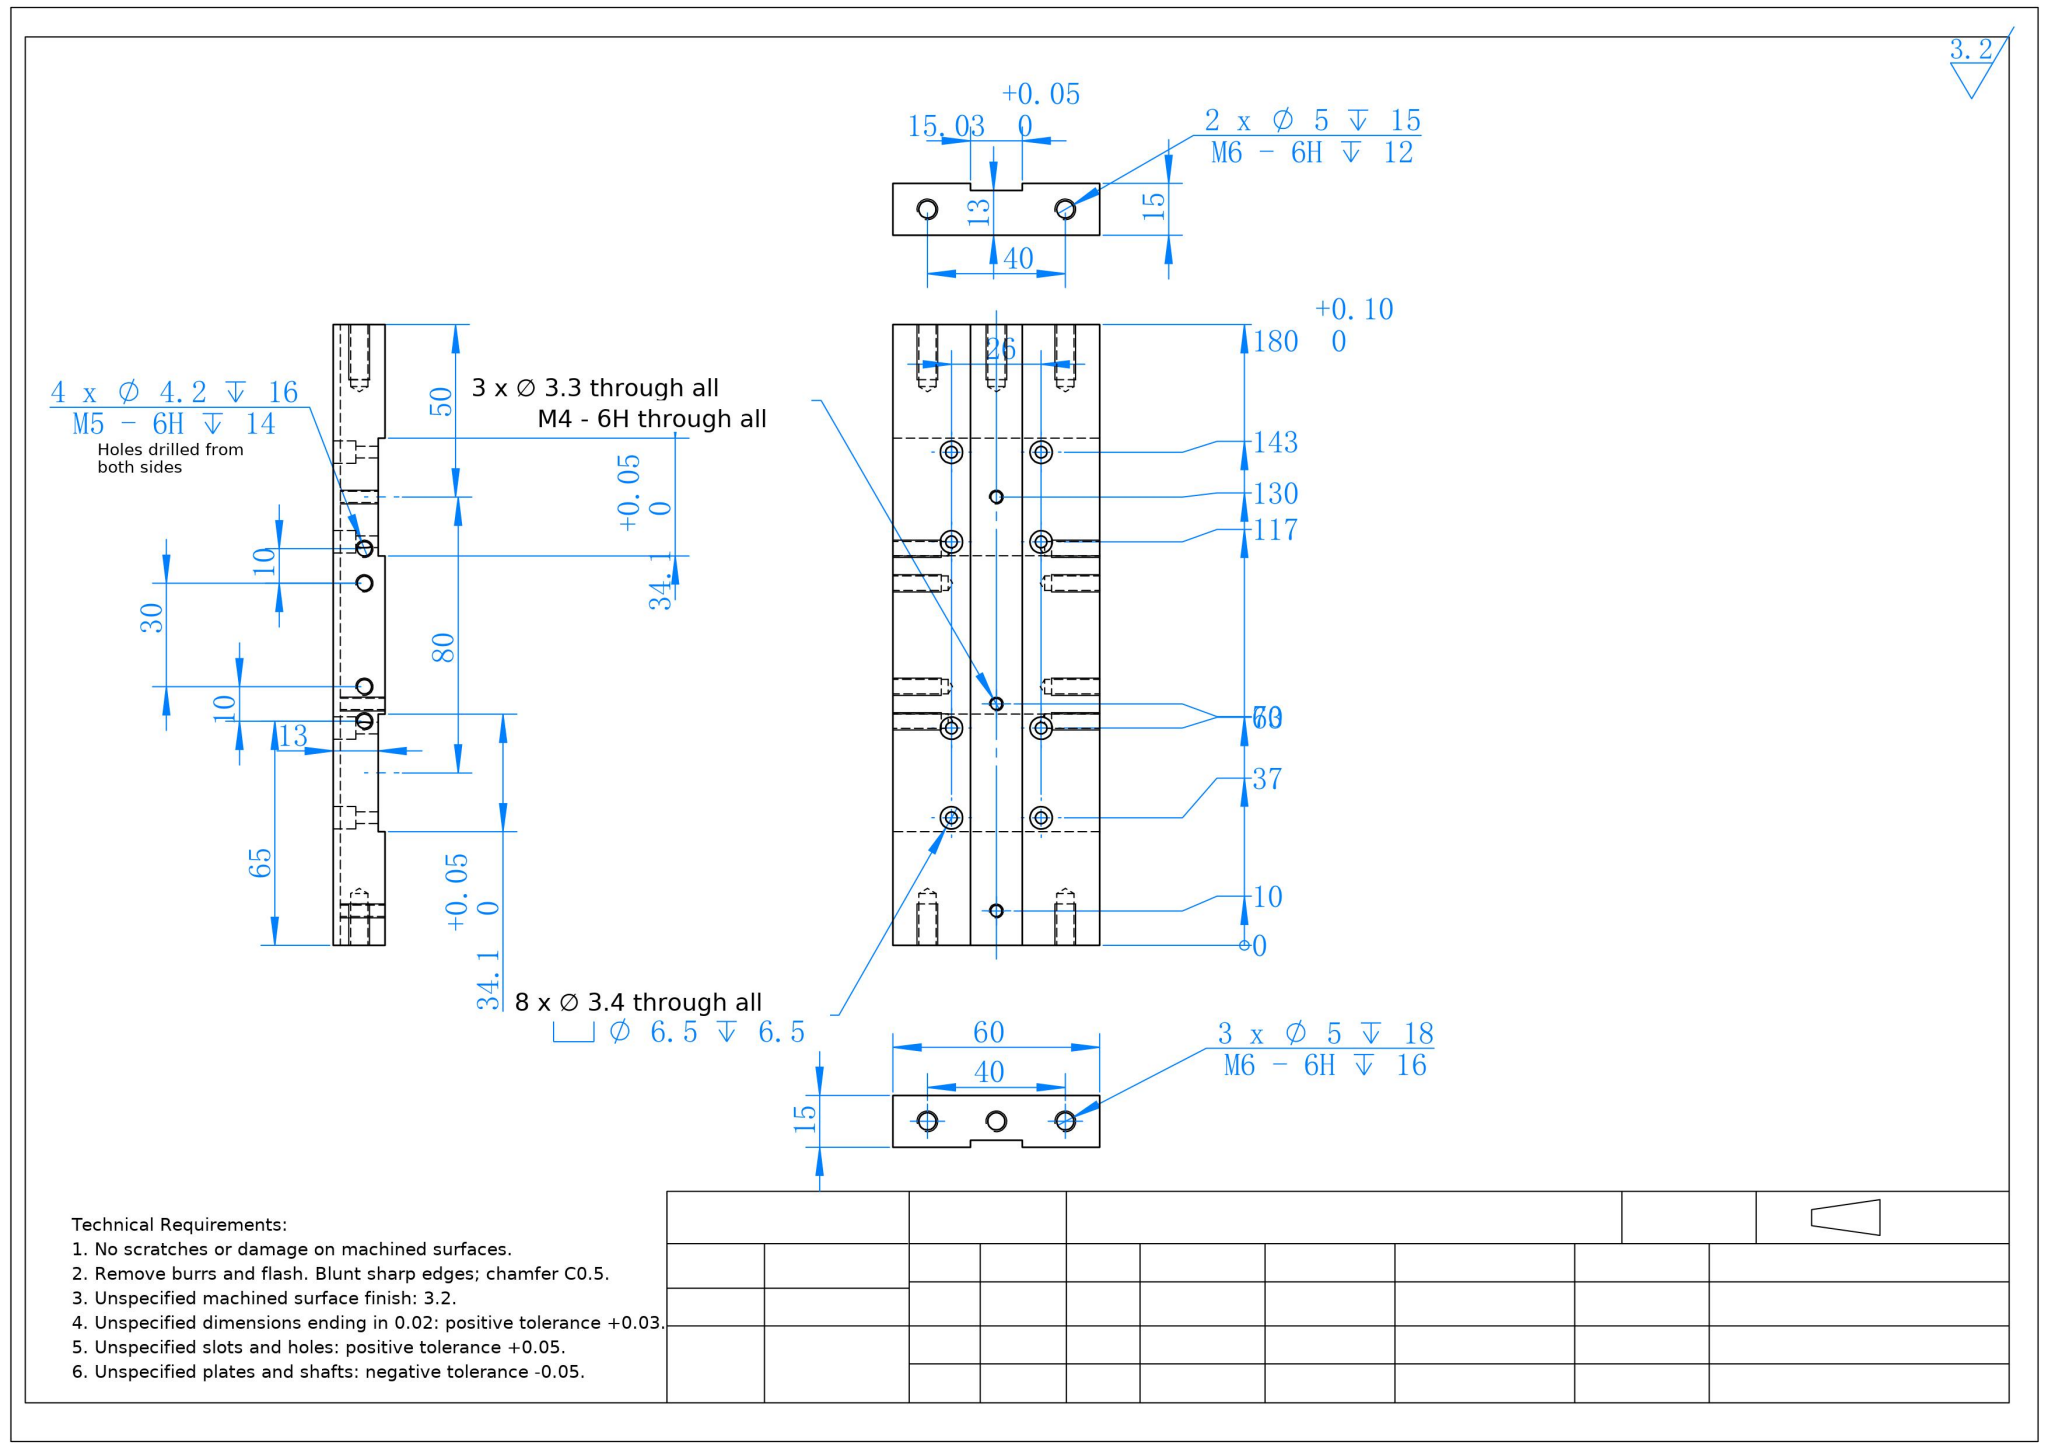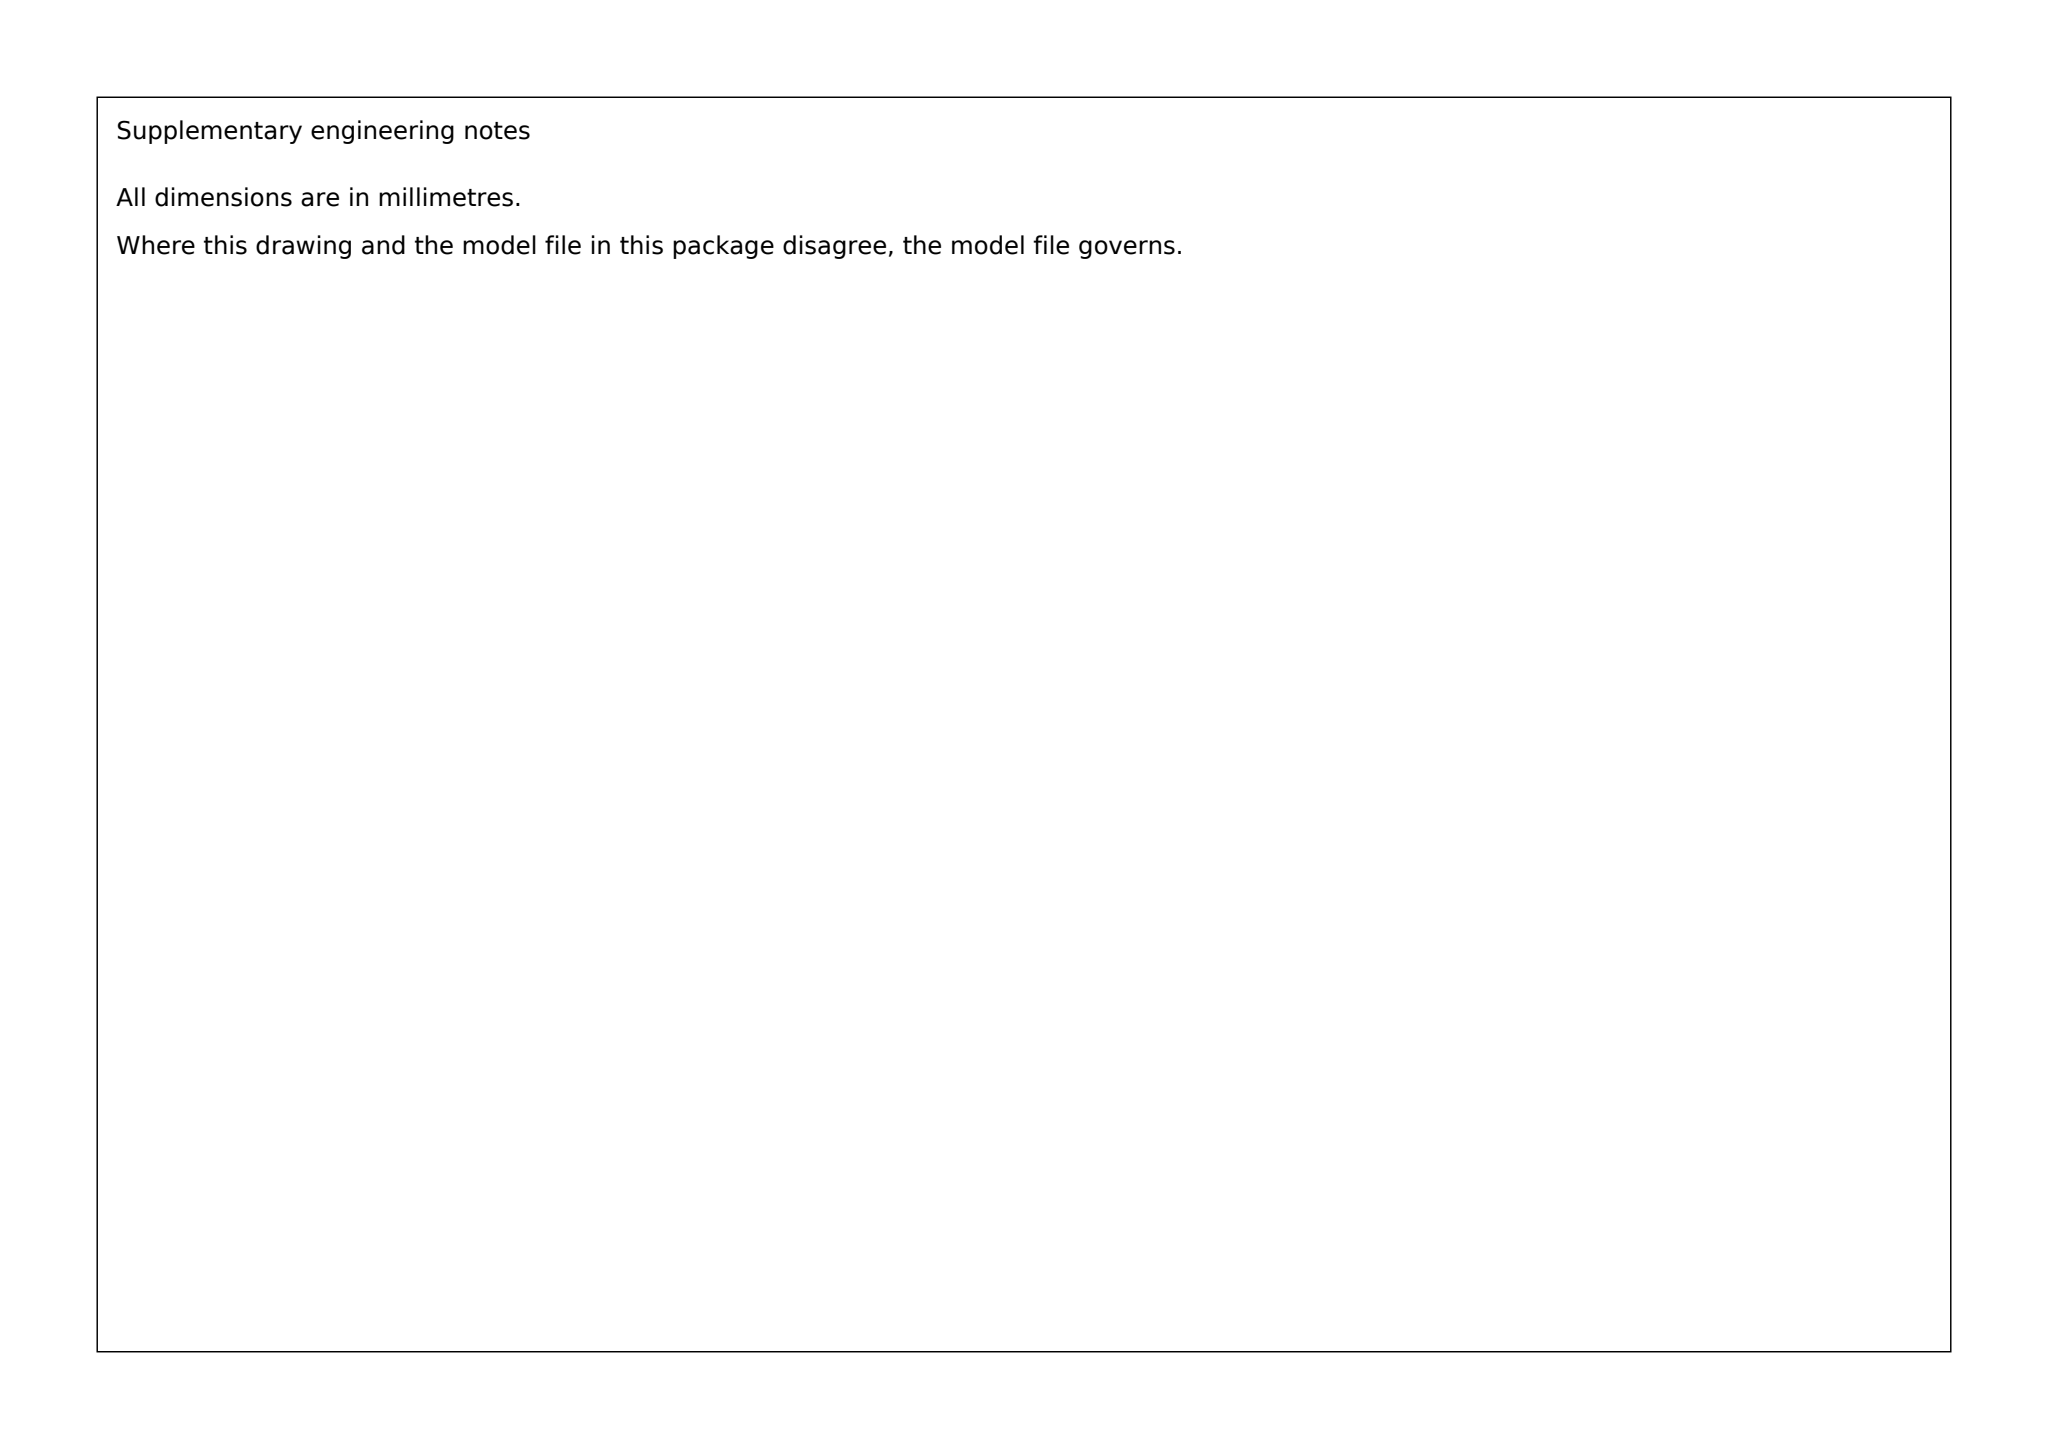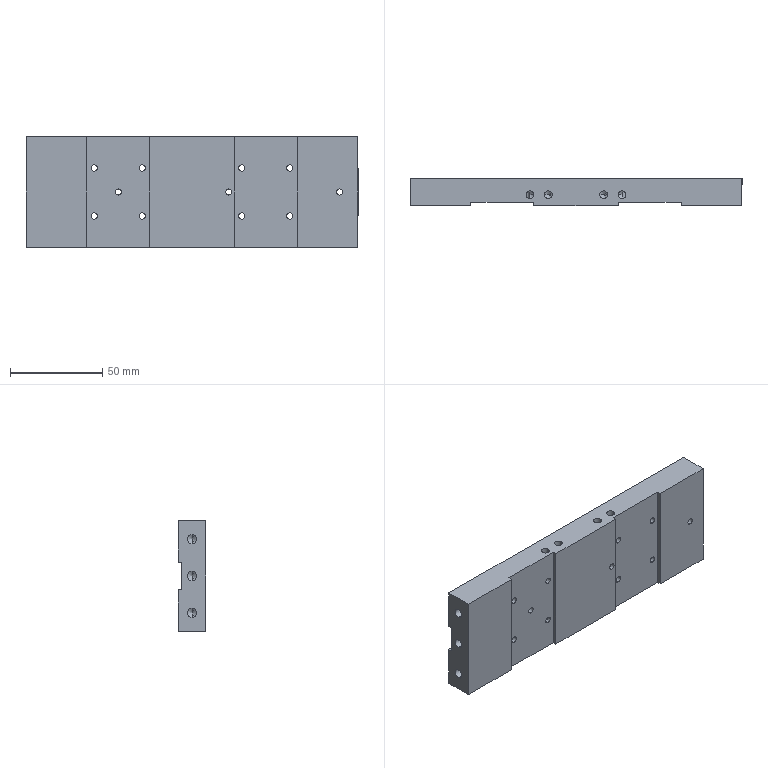Part | SolidWorks | mm | 1 solid | 116 faces | box 180 x 15 x 60 mm | volume 142388 mm3 | cylinder 64 | cone 26 | plane 26 | commonest cylinder face diameters 4.2 x16 6.5 x16 3.4 x16 5 x10 3.3 x6
build123d program:
from build123d import *

# Parameters (mm, degrees)
SKETCH1_W                                       = 180
SKETCH1_H                                       = 15
EXTRUDE1_DEPTH                                  = 30
SKETCH20_W                                      = 180
SKETCH20_H                                      = 15.03
CUT_EXTRUDE3_DEPTH                              = 2
SKETCH31_W                                      = 34.1
SKETCH31_H                                      = 60
CUT_EXTRUDE4_DEPTH                              = 2
M6_TAPPED_HOLE2_D                               = 5
M6_TAPPED_HOLE2_DEPTH                           = 18
M6_TAPPED_HOLE2_TIP                             = 1.502
M4_TAPPED_HOLE1_D                               = 3.3
M3_HEX_SOCKET_HEAD_CAP_SCREW_CBORE1_D           = 3.4
M3_HEX_SOCKET_HEAD_CAP_SCREW_CBORE1_CBORE_D     = 6.5
M3_HEX_SOCKET_HEAD_CAP_SCREW_CBORE1_CBORE_DEPTH = 6.5
M6_TAPPED_HOLE1_D                               = 5
M6_TAPPED_HOLE1_DEPTH                           = 15
M6_TAPPED_HOLE1_TIP                             = 1.502
M5_TAPPED_HOLE1_D                               = 4.2
M5_TAPPED_HOLE1_DEPTH                           = 16
M5_TAPPED_HOLE1_TIP                             = 1.262
M5_TAPPED_HOLE3_D                               = 4.2
M5_TAPPED_HOLE3_DEPTH                           = 16
M5_TAPPED_HOLE3_TIP                             = 1.262


with BuildPart() as part:
    # Sketch1 → Extrude1 (new, symmetric)
    with BuildSketch(Plane.XY):
        Rectangle(SKETCH1_W, SKETCH1_H)
    extrude(amount=EXTRUDE1_DEPTH, both=True)

    # Sketch20 → Cut-Extrude3 (cut)
    with BuildSketch(Plane(origin=(0, 7.5, 0), x_dir=(-1, 0, 0), z_dir=(0, 1, 0))):
        Rectangle(SKETCH20_W, SKETCH20_H)
    extrude(amount=-CUT_EXTRUDE3_DEPTH, mode=Mode.SUBTRACT)

    # Sketch31 → Cut-Extrude4 (cut)
    with BuildSketch(Plane(origin=(0, -7.5, 0), x_dir=(-1, 0, 0), z_dir=(0, -1, 0))):
        with Locations((40, 0)):
            Rectangle(SKETCH31_W, SKETCH31_H)
        with Locations((-40, 0)):
            Rectangle(SKETCH31_W, SKETCH31_H)
    extrude(amount=-CUT_EXTRUDE4_DEPTH, mode=Mode.SUBTRACT)

    # M6 Tapped Hole2
    with Locations(Plane.ZY.offset(90)):
        with Locations((-20, 0), (20, 0), (0, 0)):
            Hole(M6_TAPPED_HOLE2_D / 2, depth=M6_TAPPED_HOLE2_DEPTH)
            with Locations((0, 0, -(M6_TAPPED_HOLE2_DEPTH + M6_TAPPED_HOLE2_TIP / 2))):  # 118° drill point
                Cone(0, M6_TAPPED_HOLE2_D / 2, M6_TAPPED_HOLE2_TIP, mode=Mode.SUBTRACT)

    # M4 Tapped Hole1 (through all)
    with Locations(Plane(origin=(0, 7.5, 0), x_dir=(1, 0, 0), z_dir=(0, 1, 0))):
        with Locations((20, 0), (80, 0), (-40, 0)):
            Hole(M4_TAPPED_HOLE1_D / 2)

    # M3 Hex Socket Head Cap Screw CBORE1 (through all)
    with Locations(Plane(origin=(0, 7.5, 0), x_dir=(1, 0, 0), z_dir=(0, 1, 0))):
        with Locations((-53, 13), (-27, 13), (-53, -13), (-27, -13), (27, 13), (53, 13), (27, -13), (53, -13)):
            CounterBoreHole(M3_HEX_SOCKET_HEAD_CAP_SCREW_CBORE1_D / 2, M3_HEX_SOCKET_HEAD_CAP_SCREW_CBORE1_CBORE_D / 2, M3_HEX_SOCKET_HEAD_CAP_SCREW_CBORE1_CBORE_DEPTH)

    # M6 Tapped Hole1
    with Locations(Plane(origin=(90, 0, 0), x_dir=(0, 0, -1), z_dir=(1, 0, 0))):
        with Locations((-20, 0), (20, 0)):
            Hole(M6_TAPPED_HOLE1_D / 2, depth=M6_TAPPED_HOLE1_DEPTH)
            with Locations((0, 0, -(M6_TAPPED_HOLE1_DEPTH + M6_TAPPED_HOLE1_TIP / 2))):  # 118° drill point
                Cone(0, M6_TAPPED_HOLE1_D / 2, M6_TAPPED_HOLE1_TIP, mode=Mode.SUBTRACT)

    # M5 Tapped Hole1
    with Locations(Plane(origin=(0, 0, -30), x_dir=(1, 0, 0), z_dir=(0, 0, -1))):
        with Locations((-15, 1.5), (15, 1.5), (25, 1.5), (-25, 1.5)):
            Hole(M5_TAPPED_HOLE1_D / 2, depth=M5_TAPPED_HOLE1_DEPTH)
            with Locations((0, 0, -(M5_TAPPED_HOLE1_DEPTH + M5_TAPPED_HOLE1_TIP / 2))):  # 118° drill point
                Cone(0, M5_TAPPED_HOLE1_D / 2, M5_TAPPED_HOLE1_TIP, mode=Mode.SUBTRACT)

    # M5 Tapped Hole3
    with Locations(Plane.XY.offset(30)):
        with Locations((15, -1.5), (-15, -1.5), (-25, -1.5), (25, -1.5)):
            Hole(M5_TAPPED_HOLE3_D / 2, depth=M5_TAPPED_HOLE3_DEPTH)
            with Locations((0, 0, -(M5_TAPPED_HOLE3_DEPTH + M5_TAPPED_HOLE3_TIP / 2))):  # 118° drill point
                Cone(0, M5_TAPPED_HOLE3_D / 2, M5_TAPPED_HOLE3_TIP, mode=Mode.SUBTRACT)


solid = part.part